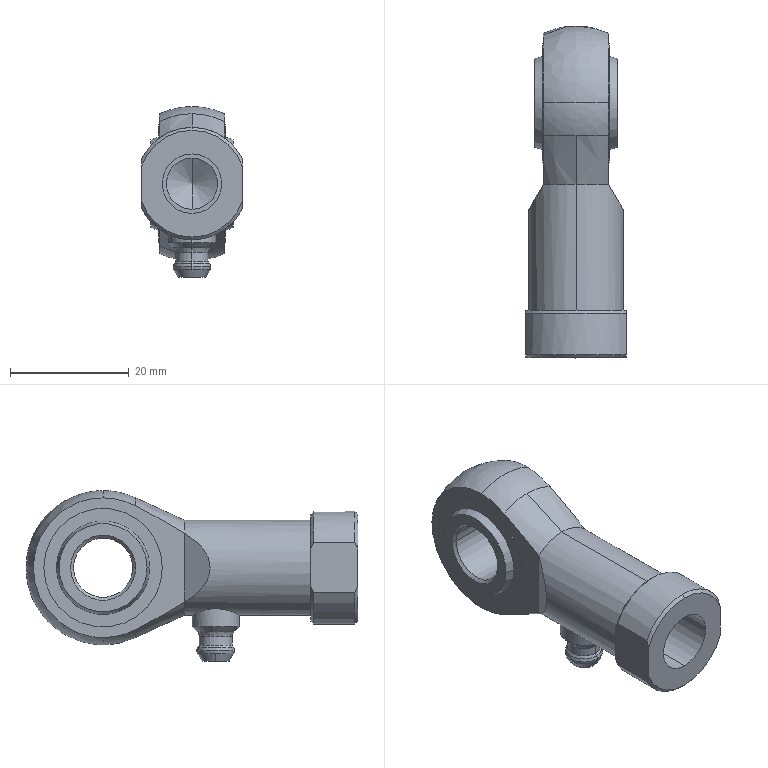Component | SolidWorks | HZ022-F-M10X125U-1 | 1 solid | 73 faces | volume 10220 mm3 | cylinder 23 | cone 21 | plane 16 | spline 13 | commonest cylinder face diameters 20 x4 19 x3 8.647 x2 10.05 x2 16 x2 8 x2 5.5 x2 10 x2 | material AL6061